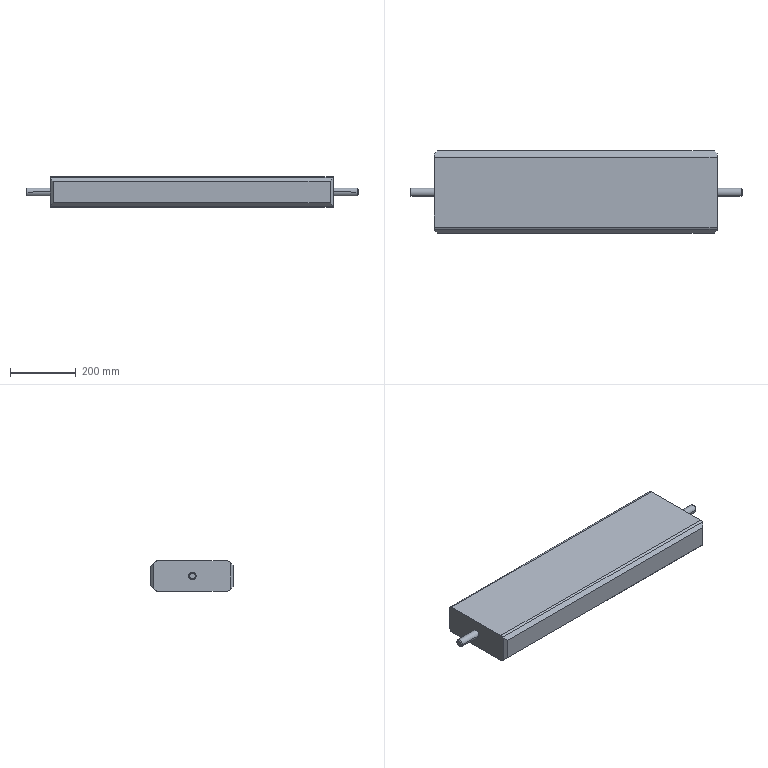Component | SolidWorks | ConnectingBeam-2 | 1 solid | 28 faces | box 1010 x 250 x 92.12 mm | volume 19465625 mm3 | plane 16 | cylinder 8 | cone 4 | commonest cylinder face diameters 24 x4 20 x4
build123d program:
from build123d import *

# Parameters (mm, degrees)
BOSS_EXTRUDE1_DEPTH              = 870
SKETCH2_2_W                      = 12
SKETCH2_2_H                      = 69
SKETCH3_2_W                      = 12
SKETCH3_2_H                      = 71
FILLET1_R                        = 10
CHAMFER1_SIZE2                   = 3
CHAMFER1_SIZE                    = 3
SKETCH2_W                        = 260
SKETCH2_H                        = 120
SKETCH2_R                        = 12
REPAIR_BEAMENDTOWEBLEFT_DEPTH    = 3
SKETCH3_W                        = 260
SKETCH3_H                        = 120
SKETCH3_R                        = 12
REPAIR_BEAMENDTOWEBRIGHT_DEPTH   = 3
REPAIR_BEAMENDCORNERRELIEF_DEPTH = 52.5


with BuildPart() as part:
    # Sketch1 → Boss-Extrude1 (new body)
    with BuildSketch(Plane.XY.offset(454.708)):
        Polygon((127.427, 230.099), (113.427, 216.099), (113.427, 151.98), (127.427, 137.98), (347.427, 137.98), (363.427, 153.98), (363.427, 214.099), (347.427, 230.099), align=None)
    extrude(amount=-BOSS_EXTRUDE1_DEPTH)

    # Sketch2_2 → Revolve1 (revolve)
    with BuildSketch(Plane.XZ.offset(-184.04), mode=Mode.PRIVATE) as revolve1_sk:
        with Locations((243.427, -449.792)):
            Rectangle(SKETCH2_2_W, SKETCH2_2_H)
    revolve(revolve1_sk.sketch.rotate(Axis((237.427, 184.04, -415.292), (0, 0, -1)), 180), axis=Axis((237.427, 184.04, -415.292), (0, 0, -1)))

    # Sketch3_2 → Revolve2 (revolve)
    with BuildSketch(Plane.XZ.offset(-184.04), mode=Mode.PRIVATE) as revolve2_sk:
        with Locations((243.427, 490.208)):
            Rectangle(SKETCH3_2_W, SKETCH3_2_H)
    revolve(revolve2_sk.sketch.rotate(Axis((237.427, 184.04, 525.708), (0, 0, -1)), 180), axis=Axis((237.427, 184.04, 525.708), (0, 0, -1)))

    # Fillet1
    fillet1_edges = [part.edges().sort_by_distance(p)[0] for p in [
        (347.427, 230.099, 19.708),
        (347.427, 137.98, 19.708),
        (127.427, 137.98, 19.708),
        (127.427, 230.099, 19.708),
    ]]
    fillet(fillet1_edges, radius=FILLET1_R)

    # Chamfer1
    chamfer1_edges = [part.edges().sort_by_distance(p)[0] for p in [
        (113.427, 184.04, -415.292),
        (249.427, 184.04, -484.292),
        (363.427, 184.04, -415.292),
        (249.427, 184.04, 525.708),
        (356.891, 220.635, -415.292),
        (237.427, 230.099, 454.708),
        (118.962, 221.635, 454.708),
        (127.742, 229.338, 454.708),
        (347.111, 229.338, 454.708),
        (237.427, 230.099, -415.292),
        (118.962, 221.635, -415.292),
        (127.742, 229.338, -415.292),
        (347.111, 229.338, -415.292),
        (356.891, 220.635, 454.708),
    ]]
    chamfer(chamfer1_edges, length=CHAMFER1_SIZE, length2=CHAMFER1_SIZE2)

    # Sketch2 → Repair_BeamEndToWebLeft (cut, symmetric)
    with BuildSketch(Plane.XY.offset(-413.292)):
        with Locations((237.427, 184.04)):
            Rectangle(SKETCH2_W, SKETCH2_H)
        with Locations(Location((237.427, 184.04, 0), (0, 0, 180))):
            Circle(SKETCH2_R, mode=Mode.SUBTRACT)
    extrude(amount=REPAIR_BEAMENDTOWEBLEFT_DEPTH, both=True, mode=Mode.SUBTRACT)

    # Sketch3 → Repair_BeamEndToWebRight (cut, symmetric)
    with BuildSketch(Plane.XY.offset(452.708)):
        with Locations((237.427, 184.04)):
            Rectangle(SKETCH3_W, SKETCH3_H)
        with Locations(Location((237.427, 184.04, 0), (0, 0, 180))):
            Circle(SKETCH3_R, mode=Mode.SUBTRACT)
    extrude(amount=REPAIR_BEAMENDTOWEBRIGHT_DEPTH, both=True, mode=Mode.SUBTRACT)

    # Sketch4 → Repair_BeamEndCornerRelief (cut, symmetric)
    with BuildSketch(Plane(origin=(0, 184.192, 0), x_dir=(1, 0, 0), z_dir=(0, 1, 0))):
        Polygon((112.427, 411.292), (112.427, 400.292), (123.427, 411.292), align=None)
        Polygon((364.427, 411.292), (364.427, 400.292), (353.427, 411.292), align=None)
        Polygon((112.427, -450.708), (112.427, -439.708), (123.427, -450.708), align=None)
        Polygon((364.427, -450.708), (364.427, -439.708), (353.427, -450.708), align=None)
    extrude(amount=REPAIR_BEAMENDCORNERRELIEF_DEPTH, both=True, mode=Mode.SUBTRACT)


solid = part.part

# Placed as in the assembly
solid = solid.moved(Location((-522.04, 1266.201, -691.692), (90, 90, 0)))
STEP:
#1=COLOUR_RGB('',0.7922,0.8196,0.9333);
#2=FILL_AREA_STYLE_COLOUR('',#1);
#3=FILL_AREA_STYLE('',(#2));
#4=SURFACE_STYLE_FILL_AREA(#3);
#5=SURFACE_SIDE_STYLE('',(#4));
#6=SURFACE_STYLE_USAGE(.BOTH.,#5);
#7=PRESENTATION_STYLE_ASSIGNMENT((#6));
#8=CARTESIAN_POINT('',(0.02629,58.725,-19.986));
#9=VERTEX_POINT('',#8);
#10=CARTESIAN_POINT('',(0.02629,59.67,-19.986));
#11=VERTEX_POINT('',#10);
#12=CARTESIAN_POINT('',(0.02629,59.198,-19.986));
#13=DIRECTION('',(-1.,0.,0.));
#14=DIRECTION('',(0.,1.,0.));
#15=AXIS2_PLACEMENT_3D('',#12,#13,#14);
#16=CIRCLE('',#15,0.4724);
#17=EDGE_CURVE('',#9,#11,#16,.T.);
#18=ORIENTED_EDGE('',*,*,#17,.T.);
#19=CARTESIAN_POINT('',(-2.848,59.67,-19.986));
#20=VERTEX_POINT('',#19);
#21=CARTESIAN_POINT('',(0.1444,59.67,-19.986));
#22=DIRECTION('',(-1.,0.,0.));
#23=VECTOR('',#22,39.37);
#24=LINE('',#21,#23);
#25=EDGE_CURVE('',#11,#20,#24,.T.);
#26=ORIENTED_EDGE('',*,*,#25,.T.);
#27=CARTESIAN_POINT('',(-2.848,58.725,-19.986));
#28=VERTEX_POINT('',#27);
#29=CARTESIAN_POINT('',(-2.848,59.198,-19.986));
#30=DIRECTION('',(1.,0.,0.));
#31=DIRECTION('',(0.,1.,0.));
#32=AXIS2_PLACEMENT_3D('',#29,#30,#31);
#33=CIRCLE('',#32,0.4724);
#34=EDGE_CURVE('',#20,#28,#33,.T.);
#35=ORIENTED_EDGE('',*,*,#34,.T.);
#36=CARTESIAN_POINT('',(0.1444,58.725,-19.986));
#37=DIRECTION('',(-1.,0.,0.));
#38=VECTOR('',#37,39.37);
#39=LINE('',#36,#38);
#40=EDGE_CURVE('',#9,#28,#39,.T.);
#41=ORIENTED_EDGE('',*,*,#40,.F.);
#42=EDGE_LOOP('',(#18,#26,#35,#41));
#43=FACE_OUTER_BOUND('',#42,.T.);
#44=CARTESIAN_POINT('',(0.1444,59.198,-19.986));
#45=DIRECTION('',(-1.,0.,0.));
#46=DIRECTION('',(0.,-1.,0.));
#47=AXIS2_PLACEMENT_3D('',#44,#45,#46);
#48=CYLINDRICAL_SURFACE('',#47,0.4724);
#49=ADVANCED_FACE('',(#43),#48,.T.);
#50=CARTESIAN_POINT('',(0.1444,59.552,-19.986));
#51=VERTEX_POINT('',#50);
#52=CARTESIAN_POINT('',(0.1444,58.844,-19.986));
#53=VERTEX_POINT('',#52);
#54=CARTESIAN_POINT('',(0.1444,59.198,-19.986));
#55=DIRECTION('',(1.,0.,0.));
#56=DIRECTION('',(0.,1.,0.));
#57=AXIS2_PLACEMENT_3D('',#54,#55,#56);
#58=CIRCLE('',#57,0.3543);
#59=EDGE_CURVE('',#51,#53,#58,.T.);
#60=ORIENTED_EDGE('',*,*,#59,.F.);
#61=CARTESIAN_POINT('',(0.02629,59.67,-19.986));
#62=DIRECTION('',(-0.7071,0.7071,0.));
#63=VECTOR('',#62,39.37);
#64=LINE('',#61,#63);
#65=EDGE_CURVE('',#51,#11,#64,.T.);
#66=ORIENTED_EDGE('',*,*,#65,.T.);
#67=ORIENTED_EDGE('',*,*,#17,.F.);
#68=CARTESIAN_POINT('',(0.02629,58.725,-19.986));
#69=DIRECTION('',(-0.7071,-0.7071,0.));
#70=VECTOR('',#69,39.37);
#71=LINE('',#68,#70);
#72=EDGE_CURVE('',#53,#9,#71,.T.);
#73=ORIENTED_EDGE('',*,*,#72,.F.);
#74=EDGE_LOOP('',(#60,#66,#67,#73));
#75=FACE_OUTER_BOUND('',#74,.T.);
#76=CARTESIAN_POINT('',(0.02629,59.198,-19.986));
#77=DIRECTION('',(-1.,0.,0.));
#78=DIRECTION('',(0.,-1.,0.));
#79=AXIS2_PLACEMENT_3D('',#76,#77,#78);
#80=CONICAL_SURFACE('',#79,0.4724,0.7854);
#81=ADVANCED_FACE('',(#75),#80,.T.);
#82=CARTESIAN_POINT('',(-36.706,59.67,-19.986));
#83=VERTEX_POINT('',#82);
#84=CARTESIAN_POINT('',(-36.706,58.725,-19.986));
#85=VERTEX_POINT('',#84);
#86=CARTESIAN_POINT('',(-36.706,59.198,-19.986));
#87=DIRECTION('',(1.,0.,0.));
#88=DIRECTION('',(0.,1.,0.));
#89=AXIS2_PLACEMENT_3D('',#86,#87,#88);
#90=CIRCLE('',#89,0.4724);
#91=EDGE_CURVE('',#83,#85,#90,.T.);
#92=ORIENTED_EDGE('',*,*,#91,.F.);
#93=CARTESIAN_POINT('',(-39.501,59.67,-19.986));
#94=VERTEX_POINT('',#93);
#95=CARTESIAN_POINT('',(-36.903,59.67,-19.986));
#96=DIRECTION('',(-1.,0.,0.));
#97=VECTOR('',#96,39.37);
#98=LINE('',#95,#97);
#99=EDGE_CURVE('',#83,#94,#98,.T.);
#100=ORIENTED_EDGE('',*,*,#99,.T.);
#101=CARTESIAN_POINT('',(-39.501,58.725,-19.986));
#102=VERTEX_POINT('',#101);
#103=CARTESIAN_POINT('',(-39.501,59.198,-19.986));
#104=DIRECTION('',(1.,0.,0.));
#105=DIRECTION('',(0.,-1.,0.));
#106=AXIS2_PLACEMENT_3D('',#103,#104,#105);
#107=CIRCLE('',#106,0.4724);
#108=EDGE_CURVE('',#94,#102,#107,.T.);
#109=ORIENTED_EDGE('',*,*,#108,.T.);
#110=CARTESIAN_POINT('',(-36.903,58.725,-19.986));
#111=DIRECTION('',(-1.,0.,0.));
#112=VECTOR('',#111,39.37);
#113=LINE('',#110,#112);
#114=EDGE_CURVE('',#85,#102,#113,.T.);
#115=ORIENTED_EDGE('',*,*,#114,.F.);
#116=EDGE_LOOP('',(#92,#100,#109,#115));
#117=FACE_OUTER_BOUND('',#116,.T.);
#118=CARTESIAN_POINT('',(-36.903,59.198,-19.986));
#119=DIRECTION('',(-1.,0.,0.));
#120=DIRECTION('',(0.,-1.,0.));
#121=AXIS2_PLACEMENT_3D('',#118,#119,#120);
#122=CYLINDRICAL_SURFACE('',#121,0.4724);
#123=ADVANCED_FACE('',(#117),#122,.T.);
#124=CARTESIAN_POINT('',(-39.619,58.844,-19.986));
#125=VERTEX_POINT('',#124);
#126=CARTESIAN_POINT('',(-39.619,59.552,-19.986));
#127=VERTEX_POINT('',#126);
#128=CARTESIAN_POINT('',(-39.619,59.198,-19.986));
#129=DIRECTION('',(-1.,0.,0.));
#130=DIRECTION('',(0.,-1.,0.));
#131=AXIS2_PLACEMENT_3D('',#128,#129,#130);
#132=CIRCLE('',#131,0.3543);
#133=EDGE_CURVE('',#125,#127,#132,.T.);
#134=ORIENTED_EDGE('',*,*,#133,.F.);
#135=CARTESIAN_POINT('',(-39.619,58.844,-19.986));
#136=DIRECTION('',(0.7071,-0.7071,0.));
#137=VECTOR('',#136,39.37);
#138=LINE('',#135,#137);
#139=EDGE_CURVE('',#125,#102,#138,.T.);
#140=ORIENTED_EDGE('',*,*,#139,.T.);
#141=ORIENTED_EDGE('',*,*,#108,.F.);
#142=CARTESIAN_POINT('',(-39.619,59.552,-19.986));
#143=DIRECTION('',(0.7071,0.7071,0.));
#144=VECTOR('',#143,39.37);
#145=LINE('',#142,#144);
#146=EDGE_CURVE('',#127,#94,#145,.T.);
#147=ORIENTED_EDGE('',*,*,#146,.F.);
#148=EDGE_LOOP('',(#134,#140,#141,#147));
#149=FACE_OUTER_BOUND('',#148,.T.);
#150=CARTESIAN_POINT('',(-39.619,59.198,-19.986));
#151=DIRECTION('',(1.,0.,0.));
#152=DIRECTION('',(0.,1.,0.));
#153=AXIS2_PLACEMENT_3D('',#150,#151,#152);
#154=CONICAL_SURFACE('',#153,0.3543,0.7854);
#155=ADVANCED_FACE('',(#149),#154,.T.);
#156=CARTESIAN_POINT('',(-36.706,55.03,-18.173));
#157=VERTEX_POINT('',#156);
#158=CARTESIAN_POINT('',(-2.848,55.03,-18.173));
#159=VERTEX_POINT('',#158);
#160=CARTESIAN_POINT('',(-36.903,55.03,-18.173));
#161=DIRECTION('',(1.,0.,0.));
#162=VECTOR('',#161,39.37);
#163=LINE('',#160,#162);
#164=EDGE_CURVE('',#157,#159,#163,.T.);
#165=ORIENTED_EDGE('',*,*,#164,.T.);
#166=CARTESIAN_POINT('',(-2.848,63.366,-18.173));
#167=VERTEX_POINT('',#166);
#168=CARTESIAN_POINT('',(-2.848,63.529,-18.173));
#169=DIRECTION('',(0.,1.,0.));
#170=VECTOR('',#169,39.37);
#171=LINE('',#168,#170);
#172=EDGE_CURVE('',#159,#167,#171,.T.);
#173=ORIENTED_EDGE('',*,*,#172,.T.);
#174=CARTESIAN_POINT('',(-36.706,63.366,-18.173));
#175=VERTEX_POINT('',#174);
#176=CARTESIAN_POINT('',(-36.903,63.366,-18.173));
#177=DIRECTION('',(-1.,0.,0.));
#178=VECTOR('',#177,39.37);
#179=LINE('',#176,#178);
#180=EDGE_CURVE('',#167,#175,#179,.T.);
#181=ORIENTED_EDGE('',*,*,#180,.T.);
#182=CARTESIAN_POINT('',(-36.706,63.529,-18.173));
#183=DIRECTION('',(0.,1.,0.));
#184=VECTOR('',#183,39.37);
#185=LINE('',#182,#184);
#186=EDGE_CURVE('',#157,#175,#185,.T.);
#187=ORIENTED_EDGE('',*,*,#186,.F.);
#188=EDGE_LOOP('',(#165,#173,#181,#187));
#189=FACE_OUTER_BOUND('',#188,.T.);
#190=CARTESIAN_POINT('',(-36.903,63.529,-18.173));
#191=DIRECTION('',(0.,0.,1.));
#192=DIRECTION('',(1.,0.,0.));
#193=AXIS2_PLACEMENT_3D('',#190,#191,#192);
#194=PLANE('',#193);
#195=ADVANCED_FACE('',(#189),#194,.T.);
#196=CARTESIAN_POINT('',(-36.706,63.804,-18.449));
#197=VERTEX_POINT('',#196);
#198=CARTESIAN_POINT('',(-36.352,64.159,-18.803));
#199=VERTEX_POINT('',#198);
#200=CARTESIAN_POINT('',(-36.535,63.975,-18.619));
#201=DIRECTION('',(0.5774,0.5774,-0.5774));
#202=VECTOR('',#201,39.37);
#203=LINE('',#200,#202);
#204=EDGE_CURVE('',#197,#199,#203,.T.);
#205=ORIENTED_EDGE('',*,*,#204,.F.);
#206=CARTESIAN_POINT('',(-36.706,63.644,-18.288));
#207=VERTEX_POINT('',#206);
#208=CARTESIAN_POINT('',(-36.706,64.159,-18.803));
#209=DIRECTION('',(0.,0.7071,-0.7071));
#210=VECTOR('',#209,39.37);
#211=LINE('',#208,#210);
#212=EDGE_CURVE('',#207,#197,#211,.T.);
#213=ORIENTED_EDGE('',*,*,#212,.F.);
#214=CARTESIAN_POINT('',(-2.848,63.644,-18.288));
#215=VERTEX_POINT('',#214);
#216=CARTESIAN_POINT('',(-36.903,63.644,-18.288));
#217=DIRECTION('',(1.,0.,0.));
#218=VECTOR('',#217,39.37);
#219=LINE('',#216,#218);
#220=EDGE_CURVE('',#207,#215,#219,.T.);
#221=ORIENTED_EDGE('',*,*,#220,.T.);
#222=CARTESIAN_POINT('',(-2.848,63.804,-18.449));
#223=VERTEX_POINT('',#222);
#224=CARTESIAN_POINT('',(-2.848,64.159,-18.803));
#225=DIRECTION('',(0.,0.7071,-0.7071));
#226=VECTOR('',#225,39.37);
#227=LINE('',#224,#226);
#228=EDGE_CURVE('',#215,#223,#227,.T.);
#229=ORIENTED_EDGE('',*,*,#228,.T.);
#230=CARTESIAN_POINT('',(-3.202,64.159,-18.803));
#231=VERTEX_POINT('',#230);
#232=CARTESIAN_POINT('',(-14.436,75.392,-30.036));
#233=DIRECTION('',(0.5774,-0.5774,0.5774));
#234=VECTOR('',#233,39.37);
#235=LINE('',#232,#234);
#236=EDGE_CURVE('',#231,#223,#235,.T.);
#237=ORIENTED_EDGE('',*,*,#236,.F.);
#238=CARTESIAN_POINT('',(-36.903,64.159,-18.803));
#239=DIRECTION('',(1.,0.,0.));
#240=VECTOR('',#239,39.37);
#241=LINE('',#238,#240);
#242=EDGE_CURVE('',#199,#231,#241,.T.);
#243=ORIENTED_EDGE('',*,*,#242,.F.);
#244=EDGE_LOOP('',(#205,#213,#221,#229,#237,#243));
#245=FACE_OUTER_BOUND('',#244,.T.);
#246=CARTESIAN_POINT('',(-36.903,64.159,-18.803));
#247=DIRECTION('',(0.,0.7071,0.7071));
#248=DIRECTION('',(0.,-0.7071,0.7071));
#249=AXIS2_PLACEMENT_3D('',#246,#247,#248);
#250=PLANE('',#249);
#251=ADVANCED_FACE('',(#245),#250,.T.);
#252=CARTESIAN_POINT('',(-36.352,64.159,-21.17));
#253=VERTEX_POINT('',#252);
#254=CARTESIAN_POINT('',(-36.352,64.159,-21.17));
#255=DIRECTION('',(0.,0.,-1.));
#256=VECTOR('',#255,39.37);
#257=LINE('',#254,#256);
#258=EDGE_CURVE('',#199,#253,#257,.T.);
#259=ORIENTED_EDGE('',*,*,#258,.F.);
#260=ORIENTED_EDGE('',*,*,#242,.T.);
#261=CARTESIAN_POINT('',(-3.202,64.159,-21.17));
#262=VERTEX_POINT('',#261);
#263=CARTESIAN_POINT('',(-3.202,64.159,-21.17));
#264=DIRECTION('',(0.,0.,1.));
#265=VECTOR('',#264,39.37);
#266=LINE('',#263,#265);
#267=EDGE_CURVE('',#262,#231,#266,.T.);
#268=ORIENTED_EDGE('',*,*,#267,.F.);
#269=CARTESIAN_POINT('',(-36.903,64.159,-21.17));
#270=DIRECTION('',(1.,0.,0.));
#271=VECTOR('',#270,39.37);
#272=LINE('',#269,#271);
#273=EDGE_CURVE('',#253,#262,#272,.T.);
#274=ORIENTED_EDGE('',*,*,#273,.F.);
#275=EDGE_LOOP('',(#259,#260,#268,#274));
#276=FACE_OUTER_BOUND('',#275,.T.);
#277=CARTESIAN_POINT('',(-36.903,64.159,-21.17));
#278=DIRECTION('',(0.,1.,0.));
#279=DIRECTION('',(-1.,0.,0.));
#280=AXIS2_PLACEMENT_3D('',#277,#278,#279);
#281=PLANE('',#280);
#282=ADVANCED_FACE('',(#276),#281,.T.);
#283=CARTESIAN_POINT('',(-36.706,63.804,-21.524));
#284=VERTEX_POINT('',#283);
#285=CARTESIAN_POINT('',(-36.955,63.555,-21.773));
#286=DIRECTION('',(-0.5774,-0.5774,-0.5774));
#287=VECTOR('',#286,39.37);
#288=LINE('',#285,#287);
#289=EDGE_CURVE('',#253,#284,#288,.T.);
#290=ORIENTED_EDGE('',*,*,#289,.F.);
#291=ORIENTED_EDGE('',*,*,#273,.T.);
#292=CARTESIAN_POINT('',(-2.848,63.804,-21.524));
#293=VERTEX_POINT('',#292);
#294=CARTESIAN_POINT('',(-14.016,74.972,-10.356));
#295=DIRECTION('',(-0.5774,0.5774,0.5774));
#296=VECTOR('',#295,39.37);
#297=LINE('',#294,#296);
#298=EDGE_CURVE('',#293,#262,#297,.T.);
#299=ORIENTED_EDGE('',*,*,#298,.F.);
#300=CARTESIAN_POINT('',(-2.848,63.644,-21.684));
#301=VERTEX_POINT('',#300);
#302=CARTESIAN_POINT('',(-2.848,63.529,-21.8));
#303=DIRECTION('',(0.,-0.7071,-0.7071));
#304=VECTOR('',#303,39.37);
#305=LINE('',#302,#304);
#306=EDGE_CURVE('',#293,#301,#305,.T.);
#307=ORIENTED_EDGE('',*,*,#306,.T.);
#308=CARTESIAN_POINT('',(-36.706,63.644,-21.684));
#309=VERTEX_POINT('',#308);
#310=CARTESIAN_POINT('',(-36.903,63.644,-21.684));
#311=DIRECTION('',(-1.,0.,0.));
#312=VECTOR('',#311,39.37);
#313=LINE('',#310,#312);
#314=EDGE_CURVE('',#301,#309,#313,.T.);
#315=ORIENTED_EDGE('',*,*,#314,.T.);
#316=CARTESIAN_POINT('',(-36.706,63.529,-21.8));
#317=DIRECTION('',(0.,-0.7071,-0.7071));
#318=VECTOR('',#317,39.37);
#319=LINE('',#316,#318);
#320=EDGE_CURVE('',#284,#309,#319,.T.);
#321=ORIENTED_EDGE('',*,*,#320,.F.);
#322=EDGE_LOOP('',(#290,#291,#299,#307,#315,#321));
#323=FACE_OUTER_BOUND('',#322,.T.);
#324=CARTESIAN_POINT('',(-36.903,63.529,-21.8));
#325=DIRECTION('',(0.,0.7071,-0.7071));
#326=DIRECTION('',(0.,0.7071,0.7071));
#327=AXIS2_PLACEMENT_3D('',#324,#325,#326);
#328=PLANE('',#327);
#329=ADVANCED_FACE('',(#323),#328,.T.);
#330=CARTESIAN_POINT('',(-36.706,63.366,-21.8));
#331=VERTEX_POINT('',#330);
#332=CARTESIAN_POINT('',(-2.848,63.366,-21.8));
#333=VERTEX_POINT('',#332);
#334=CARTESIAN_POINT('',(-36.903,63.366,-21.8));
#335=DIRECTION('',(1.,0.,0.));
#336=VECTOR('',#335,39.37);
#337=LINE('',#334,#336);
#338=EDGE_CURVE('',#331,#333,#337,.T.);
#339=ORIENTED_EDGE('',*,*,#338,.T.);
#340=CARTESIAN_POINT('',(-2.848,55.03,-21.8));
#341=VERTEX_POINT('',#340);
#342=CARTESIAN_POINT('',(-2.848,54.867,-21.8));
#343=DIRECTION('',(0.,-1.,-0.));
#344=VECTOR('',#343,39.37);
#345=LINE('',#342,#344);
#346=EDGE_CURVE('',#333,#341,#345,.T.);
#347=ORIENTED_EDGE('',*,*,#346,.T.);
#348=CARTESIAN_POINT('',(-36.706,55.03,-21.8));
#349=VERTEX_POINT('',#348);
#350=CARTESIAN_POINT('',(-36.903,55.03,-21.8));
#351=DIRECTION('',(-1.,0.,0.));
#352=VECTOR('',#351,39.37);
#353=LINE('',#350,#352);
#354=EDGE_CURVE('',#341,#349,#353,.T.);
#355=ORIENTED_EDGE('',*,*,#354,.T.);
#356=CARTESIAN_POINT('',(-36.706,54.867,-21.8));
#357=DIRECTION('',(0.,-1.,-0.));
#358=VECTOR('',#357,39.37);
#359=LINE('',#356,#358);
#360=EDGE_CURVE('',#331,#349,#359,.T.);
#361=ORIENTED_EDGE('',*,*,#360,.F.);
#362=EDGE_LOOP('',(#339,#347,#355,#361));
#363=FACE_OUTER_BOUND('',#362,.T.);
#364=CARTESIAN_POINT('',(-36.903,54.867,-21.8));
#365=DIRECTION('',(0.,0.,-1.));
#366=DIRECTION('',(0.,1.,0.));
#367=AXIS2_PLACEMENT_3D('',#364,#365,#366);
#368=PLANE('',#367);
#369=ADVANCED_FACE('',(#363),#368,.T.);
#370=CARTESIAN_POINT('',(-3.202,54.316,-21.248));
#371=VERTEX_POINT('',#370);
#372=CARTESIAN_POINT('',(-2.848,54.67,-21.603));
#373=VERTEX_POINT('',#372);
#374=CARTESIAN_POINT('',(-14.436,43.082,-10.015));
#375=DIRECTION('',(0.5774,0.5774,-0.5774));
#376=VECTOR('',#375,39.37);
#377=LINE('',#374,#376);
#378=EDGE_CURVE('',#371,#373,#377,.T.);
#379=ORIENTED_EDGE('',*,*,#378,.F.);
#380=CARTESIAN_POINT('',(-36.352,54.316,-21.248));
#381=VERTEX_POINT('',#380);
#382=CARTESIAN_POINT('',(-36.903,54.316,-21.248));
#383=DIRECTION('',(1.,0.,0.));
#384=VECTOR('',#383,39.37);
#385=LINE('',#382,#384);
#386=EDGE_CURVE('',#381,#371,#385,.T.);
#387=ORIENTED_EDGE('',*,*,#386,.F.);
#388=CARTESIAN_POINT('',(-36.706,54.67,-21.603));
#389=VERTEX_POINT('',#388);
#390=CARTESIAN_POINT('',(-36.535,54.5,-21.432));
#391=DIRECTION('',(0.5774,-0.5774,0.5774));
#392=VECTOR('',#391,39.37);
#393=LINE('',#390,#392);
#394=EDGE_CURVE('',#389,#381,#393,.T.);
#395=ORIENTED_EDGE('',*,*,#394,.F.);
#396=CARTESIAN_POINT('',(-36.706,54.752,-21.684));
#397=VERTEX_POINT('',#396);
#398=CARTESIAN_POINT('',(-36.706,54.316,-21.248));
#399=DIRECTION('',(0.,-0.7071,0.7071));
#400=VECTOR('',#399,39.37);
#401=LINE('',#398,#400);
#402=EDGE_CURVE('',#397,#389,#401,.T.);
#403=ORIENTED_EDGE('',*,*,#402,.F.);
#404=CARTESIAN_POINT('',(-2.848,54.752,-21.684));
#405=VERTEX_POINT('',#404);
#406=CARTESIAN_POINT('',(-36.903,54.752,-21.684));
#407=DIRECTION('',(1.,0.,0.));
#408=VECTOR('',#407,39.37);
#409=LINE('',#406,#408);
#410=EDGE_CURVE('',#397,#405,#409,.T.);
#411=ORIENTED_EDGE('',*,*,#410,.T.);
#412=CARTESIAN_POINT('',(-2.848,54.316,-21.248));
#413=DIRECTION('',(0.,-0.7071,0.7071));
#414=VECTOR('',#413,39.37);
#415=LINE('',#412,#414);
#416=EDGE_CURVE('',#405,#373,#415,.T.);
#417=ORIENTED_EDGE('',*,*,#416,.T.);
#418=EDGE_LOOP('',(#379,#387,#395,#403,#411,#417));
#419=FACE_OUTER_BOUND('',#418,.T.);
#420=CARTESIAN_POINT('',(-36.903,54.316,-21.248));
#421=DIRECTION('',(0.,-0.7071,-0.7071));
#422=DIRECTION('',(0.,0.7071,-0.7071));
#423=AXIS2_PLACEMENT_3D('',#420,#421,#422);
#424=PLANE('',#423);
#425=ADVANCED_FACE('',(#419),#424,.T.);
#426=CARTESIAN_POINT('',(-3.202,54.316,-18.724));
#427=VERTEX_POINT('',#426);
#428=CARTESIAN_POINT('',(-3.202,54.316,-18.724));
#429=DIRECTION('',(0.,0.,-1.));
#430=VECTOR('',#429,39.37);
#431=LINE('',#428,#430);
#432=EDGE_CURVE('',#427,#371,#431,.T.);
#433=ORIENTED_EDGE('',*,*,#432,.F.);
#434=CARTESIAN_POINT('',(-36.352,54.316,-18.724));
#435=VERTEX_POINT('',#434);
#436=CARTESIAN_POINT('',(-36.903,54.316,-18.724));
#437=DIRECTION('',(1.,0.,0.));
#438=VECTOR('',#437,39.37);
#439=LINE('',#436,#438);
#440=EDGE_CURVE('',#435,#427,#439,.T.);
#441=ORIENTED_EDGE('',*,*,#440,.F.);
#442=CARTESIAN_POINT('',(-36.352,54.316,-18.724));
#443=DIRECTION('',(0.,0.,1.));
#444=VECTOR('',#443,39.37);
#445=LINE('',#442,#444);
#446=EDGE_CURVE('',#381,#435,#445,.T.);
#447=ORIENTED_EDGE('',*,*,#446,.F.);
#448=ORIENTED_EDGE('',*,*,#386,.T.);
#449=EDGE_LOOP('',(#433,#441,#447,#448));
#450=FACE_OUTER_BOUND('',#449,.T.);
#451=CARTESIAN_POINT('',(-36.903,54.316,-18.724));
#452=DIRECTION('',(0.,-1.,0.));
#453=DIRECTION('',(1.,0.,0.));
#454=AXIS2_PLACEMENT_3D('',#451,#452,#453);
#455=PLANE('',#454);
#456=ADVANCED_FACE('',(#450),#455,.T.);
#457=CARTESIAN_POINT('',(-2.848,54.67,-18.37));
#458=VERTEX_POINT('',#457);
#459=CARTESIAN_POINT('',(-14.068,43.45,-29.59));
#460=DIRECTION('',(-0.5774,-0.5774,-0.5774));
#461=VECTOR('',#460,39.37);
#462=LINE('',#459,#461);
#463=EDGE_CURVE('',#458,#427,#462,.T.);
#464=ORIENTED_EDGE('',*,*,#463,.F.);
#465=CARTESIAN_POINT('',(-2.848,54.752,-18.288));
#466=VERTEX_POINT('',#465);
#467=CARTESIAN_POINT('',(-2.848,54.867,-18.173));
#468=DIRECTION('',(0.,0.7071,0.7071));
#469=VECTOR('',#468,39.37);
#470=LINE('',#467,#469);
#471=EDGE_CURVE('',#458,#466,#470,.T.);
#472=ORIENTED_EDGE('',*,*,#471,.T.);
#473=CARTESIAN_POINT('',(-36.706,54.752,-18.288));
#474=VERTEX_POINT('',#473);
#475=CARTESIAN_POINT('',(-36.903,54.752,-18.288));
#476=DIRECTION('',(-1.,0.,0.));
#477=VECTOR('',#476,39.37);
#478=LINE('',#475,#477);
#479=EDGE_CURVE('',#466,#474,#478,.T.);
#480=ORIENTED_EDGE('',*,*,#479,.T.);
#481=CARTESIAN_POINT('',(-36.706,54.67,-18.37));
#482=VERTEX_POINT('',#481);
#483=CARTESIAN_POINT('',(-36.706,54.867,-18.173));
#484=DIRECTION('',(0.,0.7071,0.7071));
#485=VECTOR('',#484,39.37);
#486=LINE('',#483,#485);
#487=EDGE_CURVE('',#482,#474,#486,.T.);
#488=ORIENTED_EDGE('',*,*,#487,.F.);
#489=CARTESIAN_POINT('',(-36.903,54.867,-18.173));
#490=DIRECTION('',(-0.5774,0.5774,0.5774));
#491=VECTOR('',#490,39.37);
#492=LINE('',#489,#491);
#493=EDGE_CURVE('',#435,#482,#492,.T.);
#494=ORIENTED_EDGE('',*,*,#493,.F.);
#495=ORIENTED_EDGE('',*,*,#440,.T.);
#496=EDGE_LOOP('',(#464,#472,#480,#488,#494,#495));
#497=FACE_OUTER_BOUND('',#496,.T.);
#498=CARTESIAN_POINT('',(-36.903,54.867,-18.173));
#499=DIRECTION('',(0.,-0.7071,0.7071));
#500=DIRECTION('',(0.,-0.7071,-0.7071));
#501=AXIS2_PLACEMENT_3D('',#498,#499,#500);
#502=PLANE('',#501);
#503=ADVANCED_FACE('',(#497),#502,.T.);
#504=ORIENTED_EDGE('',*,*,#314,.F.);
#505=CARTESIAN_POINT('',(-2.848,63.366,-21.406));
#506=DIRECTION('',(-1.,0.,0.));
#507=DIRECTION('',(0.,1.,0.));
#508=AXIS2_PLACEMENT_3D('',#505,#506,#507);
#509=CIRCLE('',#508,0.3937);
#510=EDGE_CURVE('',#301,#333,#509,.T.);
#511=ORIENTED_EDGE('',*,*,#510,.T.);
#512=ORIENTED_EDGE('',*,*,#338,.F.);
#513=CARTESIAN_POINT('',(-36.706,63.366,-21.406));
#514=DIRECTION('',(-1.,0.,0.));
#515=DIRECTION('',(0.,1.,0.));
#516=AXIS2_PLACEMENT_3D('',#513,#514,#515);
#517=CIRCLE('',#516,0.3937);
#518=EDGE_CURVE('',#309,#331,#517,.T.);
#519=ORIENTED_EDGE('',*,*,#518,.F.);
#520=EDGE_LOOP('',(#504,#511,#512,#519));
#521=FACE_OUTER_BOUND('',#520,.T.);
#522=CARTESIAN_POINT('',(-36.903,63.366,-21.406));
#523=DIRECTION('',(1.,0.,0.));
#524=DIRECTION('',(0.,1.,0.));
#525=AXIS2_PLACEMENT_3D('',#522,#523,#524);
#526=CYLINDRICAL_SURFACE('',#525,0.3937);
#527=ADVANCED_FACE('',(#521),#526,.T.);
#528=ORIENTED_EDGE('',*,*,#354,.F.);
#529=CARTESIAN_POINT('',(-2.848,55.03,-21.406));
#530=DIRECTION('',(-1.,0.,0.));
#531=DIRECTION('',(0.,1.,0.));
#532=AXIS2_PLACEMENT_3D('',#529,#530,#531);
#533=CIRCLE('',#532,0.3937);
#534=EDGE_CURVE('',#341,#405,#533,.T.);
#535=ORIENTED_EDGE('',*,*,#534,.T.);
#536=ORIENTED_EDGE('',*,*,#410,.F.);
#537=CARTESIAN_POINT('',(-36.706,55.03,-21.406));
#538=DIRECTION('',(-1.,0.,0.));
#539=DIRECTION('',(0.,1.,0.));
#540=AXIS2_PLACEMENT_3D('',#537,#538,#539);
#541=CIRCLE('',#540,0.3937);
#542=EDGE_CURVE('',#349,#397,#541,.T.);
#543=ORIENTED_EDGE('',*,*,#542,.F.);
#544=EDGE_LOOP('',(#528,#535,#536,#543));
#545=FACE_OUTER_BOUND('',#544,.T.);
#546=CARTESIAN_POINT('',(-36.903,55.03,-21.406));
#547=DIRECTION('',(1.,0.,0.));
#548=DIRECTION('',(0.,1.,0.));
#549=AXIS2_PLACEMENT_3D('',#546,#547,#548);
#550=CYLINDRICAL_SURFACE('',#549,0.3937);
#551=ADVANCED_FACE('',(#545),#550,.T.);
#552=ORIENTED_EDGE('',*,*,#180,.F.);
#553=CARTESIAN_POINT('',(-2.848,63.366,-18.567));
#554=DIRECTION('',(-1.,0.,0.));
#555=DIRECTION('',(0.,1.,-0.));
#556=AXIS2_PLACEMENT_3D('',#553,#554,#555);
#557=CIRCLE('',#556,0.3937);
#558=EDGE_CURVE('',#167,#215,#557,.T.);
#559=ORIENTED_EDGE('',*,*,#558,.T.);
#560=ORIENTED_EDGE('',*,*,#220,.F.);
#561=CARTESIAN_POINT('',(-36.706,63.366,-18.567));
#562=DIRECTION('',(-1.,0.,0.));
#563=DIRECTION('',(0.,1.,-0.));
#564=AXIS2_PLACEMENT_3D('',#561,#562,#563);
#565=CIRCLE('',#564,0.3937);
#566=EDGE_CURVE('',#175,#207,#565,.T.);
#567=ORIENTED_EDGE('',*,*,#566,.F.);
#568=EDGE_LOOP('',(#552,#559,#560,#567));
#569=FACE_OUTER_BOUND('',#568,.T.);
#570=CARTESIAN_POINT('',(-36.903,63.366,-18.567));
#571=DIRECTION('',(1.,0.,0.));
#572=DIRECTION('',(0.,1.,0.));
#573=AXIS2_PLACEMENT_3D('',#570,#571,#572);
#574=CYLINDRICAL_SURFACE('',#573,0.3937);
#575=ADVANCED_FACE('',(#569),#574,.T.);
#576=ORIENTED_EDGE('',*,*,#479,.F.);
#577=CARTESIAN_POINT('',(-2.848,55.03,-18.567));
#578=DIRECTION('',(-1.,0.,0.));
#579=DIRECTION('',(0.,1.,-0.));
#580=AXIS2_PLACEMENT_3D('',#577,#578,#579);
#581=CIRCLE('',#580,0.3937);
#582=EDGE_CURVE('',#466,#159,#581,.T.);
#583=ORIENTED_EDGE('',*,*,#582,.T.);
#584=ORIENTED_EDGE('',*,*,#164,.F.);
#585=CARTESIAN_POINT('',(-36.706,55.03,-18.567));
#586=DIRECTION('',(-1.,0.,0.));
#587=DIRECTION('',(0.,1.,-0.));
#588=AXIS2_PLACEMENT_3D('',#585,#586,#587);
#589=CIRCLE('',#588,0.3937);
#590=EDGE_CURVE('',#474,#157,#589,.T.);
#591=ORIENTED_EDGE('',*,*,#590,.F.);
#592=EDGE_LOOP('',(#576,#583,#584,#591));
#593=FACE_OUTER_BOUND('',#592,.T.);
#594=CARTESIAN_POINT('',(-36.903,55.03,-18.567));
#595=DIRECTION('',(1.,0.,0.));
#596=DIRECTION('',(0.,1.,0.));
#597=AXIS2_PLACEMENT_3D('',#594,#595,#596);
#598=CYLINDRICAL_SURFACE('',#597,0.3937);
#599=ADVANCED_FACE('',(#593),#598,.T.);
#600=ORIENTED_EDGE('',*,*,#212,.T.);
#601=CARTESIAN_POINT('',(-36.706,63.804,-27.232));
#602=DIRECTION('',(0.,0.,-1.));
#603=VECTOR('',#602,39.37);
#604=LINE('',#601,#603);
#605=EDGE_CURVE('',#197,#284,#604,.T.);
#606=ORIENTED_EDGE('',*,*,#605,.T.);
#607=ORIENTED_EDGE('',*,*,#320,.T.);
#608=ORIENTED_EDGE('',*,*,#518,.T.);
#609=ORIENTED_EDGE('',*,*,#360,.T.);
#610=ORIENTED_EDGE('',*,*,#542,.T.);
#611=ORIENTED_EDGE('',*,*,#402,.T.);
#612=CARTESIAN_POINT('',(-36.706,54.67,-27.232));
#613=DIRECTION('',(0.,0.,1.));
#614=VECTOR('',#613,39.37);
#615=LINE('',#612,#614);
#616=EDGE_CURVE('',#389,#482,#615,.T.);
#617=ORIENTED_EDGE('',*,*,#616,.T.);
#618=ORIENTED_EDGE('',*,*,#487,.T.);
#619=ORIENTED_EDGE('',*,*,#590,.T.);
#620=ORIENTED_EDGE('',*,*,#186,.T.);
#621=ORIENTED_EDGE('',*,*,#566,.T.);
#622=EDGE_LOOP('',(#600,#606,#607,#608,#609,#610,#611,#617,#618,#619,#620,#621));
#623=FACE_OUTER_BOUND('',#622,.T.);
#624=CARTESIAN_POINT('',(-36.706,59.198,-19.986));
#625=DIRECTION('',(1.,0.,0.));
#626=DIRECTION('',(0.,1.,0.));
#627=AXIS2_PLACEMENT_3D('',#624,#625,#626);
#628=CIRCLE('',#627,0.4724);
#629=EDGE_CURVE('',#85,#83,#628,.T.);
#630=ORIENTED_EDGE('',*,*,#629,.T.);
#631=ORIENTED_EDGE('',*,*,#91,.T.);
#632=EDGE_LOOP('',(#630,#631));
#633=FACE_BOUND('',#632,.T.);
#634=CARTESIAN_POINT('',(-36.706,49.85,-27.232));
#635=DIRECTION('',(1.,0.,0.));
#636=DIRECTION('',(0.,1.,0.));
#637=AXIS2_PLACEMENT_3D('',#634,#635,#636);
#638=PLANE('',#637);
#639=ADVANCED_FACE('',(#623,#633),#638,.F.);
#640=CARTESIAN_POINT('',(-39.619,59.198,-19.986));
#641=DIRECTION('',(-1.,0.,0.));
#642=DIRECTION('',(0.,-1.,0.));
#643=AXIS2_PLACEMENT_3D('',#640,#641,#642);
#644=CIRCLE('',#643,0.3543);
#645=EDGE_CURVE('',#127,#125,#644,.T.);
#646=ORIENTED_EDGE('',*,*,#645,.T.);
#647=ORIENTED_EDGE('',*,*,#133,.T.);
#648=EDGE_LOOP('',(#646,#647));
#649=FACE_OUTER_BOUND('',#648,.T.);
#650=CARTESIAN_POINT('',(-39.619,59.198,-19.986));
#651=DIRECTION('',(-1.,0.,0.));
#652=DIRECTION('',(0.,-1.,0.));
#653=AXIS2_PLACEMENT_3D('',#650,#651,#652);
#654=PLANE('',#653);
#655=ADVANCED_FACE('',(#649),#654,.T.);
#656=ORIENTED_EDGE('',*,*,#139,.F.);
#657=ORIENTED_EDGE('',*,*,#645,.F.);
#658=ORIENTED_EDGE('',*,*,#146,.T.);
#659=CARTESIAN_POINT('',(-39.501,59.198,-19.986));
#660=DIRECTION('',(1.,0.,0.));
#661=DIRECTION('',(0.,-1.,0.));
#662=AXIS2_PLACEMENT_3D('',#659,#660,#661);
#663=CIRCLE('',#662,0.4724);
#664=EDGE_CURVE('',#102,#94,#663,.T.);
#665=ORIENTED_EDGE('',*,*,#664,.F.);
#666=EDGE_LOOP('',(#656,#657,#658,#665));
#667=FACE_OUTER_BOUND('',#666,.T.);
#668=CARTESIAN_POINT('',(-39.619,59.198,-19.986));
#669=DIRECTION('',(1.,0.,0.));
#670=DIRECTION('',(0.,1.,0.));
#671=AXIS2_PLACEMENT_3D('',#668,#669,#670);
#672=CONICAL_SURFACE('',#671,0.3543,0.7854);
#673=ADVANCED_FACE('',(#667),#672,.T.);
#674=ORIENTED_EDGE('',*,*,#99,.F.);
#675=ORIENTED_EDGE('',*,*,#629,.F.);
#676=ORIENTED_EDGE('',*,*,#114,.T.);
#677=ORIENTED_EDGE('',*,*,#664,.T.);
#678=EDGE_LOOP('',(#674,#675,#676,#677));
#679=FACE_OUTER_BOUND('',#678,.T.);
#680=CARTESIAN_POINT('',(-36.903,59.198,-19.986));
#681=DIRECTION('',(-1.,0.,0.));
#682=DIRECTION('',(0.,-1.,0.));
#683=AXIS2_PLACEMENT_3D('',#680,#681,#682);
#684=CYLINDRICAL_SURFACE('',#683,0.4724);
#685=ADVANCED_FACE('',(#679),#684,.T.);
#686=CARTESIAN_POINT('',(-2.848,54.67,-27.232));
#687=DIRECTION('',(0.,0.,1.));
#688=VECTOR('',#687,39.37);
#689=LINE('',#686,#688);
#690=EDGE_CURVE('',#373,#458,#689,.T.);
#691=ORIENTED_EDGE('',*,*,#690,.F.);
#692=ORIENTED_EDGE('',*,*,#416,.F.);
#693=ORIENTED_EDGE('',*,*,#534,.F.);
#694=ORIENTED_EDGE('',*,*,#346,.F.);
#695=ORIENTED_EDGE('',*,*,#510,.F.);
#696=ORIENTED_EDGE('',*,*,#306,.F.);
#697=CARTESIAN_POINT('',(-2.848,63.804,-27.232));
#698=DIRECTION('',(0.,0.,-1.));
#699=VECTOR('',#698,39.37);
#700=LINE('',#697,#699);
#701=EDGE_CURVE('',#223,#293,#700,.T.);
#702=ORIENTED_EDGE('',*,*,#701,.F.);
#703=ORIENTED_EDGE('',*,*,#228,.F.);
#704=ORIENTED_EDGE('',*,*,#558,.F.);
#705=ORIENTED_EDGE('',*,*,#172,.F.);
#706=ORIENTED_EDGE('',*,*,#582,.F.);
#707=ORIENTED_EDGE('',*,*,#471,.F.);
#708=EDGE_LOOP('',(#691,#692,#693,#694,#695,#696,#702,#703,#704,#705,#706,#707));
#709=FACE_OUTER_BOUND('',#708,.T.);
#710=CARTESIAN_POINT('',(-2.848,59.198,-19.986));
#711=DIRECTION('',(1.,0.,0.));
#712=DIRECTION('',(0.,1.,0.));
#713=AXIS2_PLACEMENT_3D('',#710,#711,#712);
#714=CIRCLE('',#713,0.4724);
#715=EDGE_CURVE('',#28,#20,#714,.T.);
#716=ORIENTED_EDGE('',*,*,#715,.F.);
#717=ORIENTED_EDGE('',*,*,#34,.F.);
#718=EDGE_LOOP('',(#716,#717));
#719=FACE_BOUND('',#718,.T.);
#720=CARTESIAN_POINT('',(-2.848,49.85,-27.232));
#721=DIRECTION('',(1.,0.,0.));
#722=DIRECTION('',(0.,1.,0.));
#723=AXIS2_PLACEMENT_3D('',#720,#721,#722);
#724=PLANE('',#723);
#725=ADVANCED_FACE('',(#709,#719),#724,.T.);
#726=CARTESIAN_POINT('',(0.1444,59.198,-19.986));
#727=DIRECTION('',(1.,0.,0.));
#728=DIRECTION('',(0.,1.,0.));
#729=AXIS2_PLACEMENT_3D('',#726,#727,#728);
#730=CIRCLE('',#729,0.3543);
#731=EDGE_CURVE('',#53,#51,#730,.T.);
#732=ORIENTED_EDGE('',*,*,#731,.T.);
#733=ORIENTED_EDGE('',*,*,#59,.T.);
#734=EDGE_LOOP('',(#732,#733));
#735=FACE_OUTER_BOUND('',#734,.T.);
#736=CARTESIAN_POINT('',(0.1444,59.67,-19.986));
#737=DIRECTION('',(1.,0.,0.));
#738=DIRECTION('',(0.,1.,0.));
#739=AXIS2_PLACEMENT_3D('',#736,#737,#738);
#740=PLANE('',#739);
#741=ADVANCED_FACE('',(#735),#740,.T.);
#742=ORIENTED_EDGE('',*,*,#65,.F.);
#743=ORIENTED_EDGE('',*,*,#731,.F.);
#744=ORIENTED_EDGE('',*,*,#72,.T.);
#745=CARTESIAN_POINT('',(0.02629,59.198,-19.986));
#746=DIRECTION('',(-1.,0.,0.));
#747=DIRECTION('',(0.,1.,0.));
#748=AXIS2_PLACEMENT_3D('',#745,#746,#747);
#749=CIRCLE('',#748,0.4724);
#750=EDGE_CURVE('',#11,#9,#749,.T.);
#751=ORIENTED_EDGE('',*,*,#750,.F.);
#752=EDGE_LOOP('',(#742,#743,#744,#751));
#753=FACE_OUTER_BOUND('',#752,.T.);
#754=CARTESIAN_POINT('',(0.02629,59.198,-19.986));
#755=DIRECTION('',(-1.,0.,0.));
#756=DIRECTION('',(0.,-1.,0.));
#757=AXIS2_PLACEMENT_3D('',#754,#755,#756);
#758=CONICAL_SURFACE('',#757,0.4724,0.7854);
#759=ADVANCED_FACE('',(#753),#758,.T.);
#760=ORIENTED_EDGE('',*,*,#25,.F.);
#761=ORIENTED_EDGE('',*,*,#750,.T.);
#762=ORIENTED_EDGE('',*,*,#40,.T.);
#763=ORIENTED_EDGE('',*,*,#715,.T.);
#764=EDGE_LOOP('',(#760,#761,#762,#763));
#765=FACE_OUTER_BOUND('',#764,.T.);
#766=CARTESIAN_POINT('',(0.1444,59.198,-19.986));
#767=DIRECTION('',(-1.,0.,0.));
#768=DIRECTION('',(0.,-1.,0.));
#769=AXIS2_PLACEMENT_3D('',#766,#767,#768);
#770=CYLINDRICAL_SURFACE('',#769,0.4724);
#771=ADVANCED_FACE('',(#765),#770,.T.);
#772=ORIENTED_EDGE('',*,*,#236,.T.);
#773=ORIENTED_EDGE('',*,*,#701,.T.);
#774=ORIENTED_EDGE('',*,*,#298,.T.);
#775=ORIENTED_EDGE('',*,*,#267,.T.);
#776=EDGE_LOOP('',(#772,#773,#774,#775));
#777=FACE_OUTER_BOUND('',#776,.T.);
#778=CARTESIAN_POINT('',(-3.241,64.198,-22.047));
#779=DIRECTION('',(-0.7071,-0.7071,0.));
#780=DIRECTION('',(0.7071,-0.7071,0.));
#781=AXIS2_PLACEMENT_3D('',#778,#779,#780);
#782=PLANE('',#781);
#783=ADVANCED_FACE('',(#777),#782,.F.);
#784=ORIENTED_EDGE('',*,*,#378,.T.);
#785=ORIENTED_EDGE('',*,*,#690,.T.);
#786=ORIENTED_EDGE('',*,*,#463,.T.);
#787=ORIENTED_EDGE('',*,*,#432,.T.);
#788=EDGE_LOOP('',(#784,#785,#786,#787));
#789=FACE_OUTER_BOUND('',#788,.T.);
#790=CARTESIAN_POINT('',(-3.241,54.277,-22.047));
#791=DIRECTION('',(-0.7071,0.7071,0.));
#792=DIRECTION('',(-0.7071,-0.7071,0.));
#793=AXIS2_PLACEMENT_3D('',#790,#791,#792);
#794=PLANE('',#793);
#795=ADVANCED_FACE('',(#789),#794,.F.);
#796=ORIENTED_EDGE('',*,*,#394,.T.);
#797=ORIENTED_EDGE('',*,*,#446,.T.);
#798=ORIENTED_EDGE('',*,*,#493,.T.);
#799=ORIENTED_EDGE('',*,*,#616,.F.);
#800=EDGE_LOOP('',(#796,#797,#798,#799));
#801=FACE_OUTER_BOUND('',#800,.T.);
#802=CARTESIAN_POINT('',(-36.312,54.277,-22.047));
#803=DIRECTION('',(0.7071,0.7071,0.));
#804=DIRECTION('',(-0.7071,0.7071,0.));
#805=AXIS2_PLACEMENT_3D('',#802,#803,#804);
#806=PLANE('',#805);
#807=ADVANCED_FACE('',(#801),#806,.F.);
#808=ORIENTED_EDGE('',*,*,#204,.T.);
#809=ORIENTED_EDGE('',*,*,#258,.T.);
#810=ORIENTED_EDGE('',*,*,#289,.T.);
#811=ORIENTED_EDGE('',*,*,#605,.F.);
#812=EDGE_LOOP('',(#808,#809,#810,#811));
#813=FACE_OUTER_BOUND('',#812,.T.);
#814=CARTESIAN_POINT('',(-36.312,64.198,-22.047));
#815=DIRECTION('',(0.7071,-0.7071,0.));
#816=DIRECTION('',(0.7071,0.7071,0.));
#817=AXIS2_PLACEMENT_3D('',#814,#815,#816);
#818=PLANE('',#817);
#819=ADVANCED_FACE('',(#813),#818,.F.);
#820=CLOSED_SHELL('',(#49,#81,#123,#155,#195,#251,#282,#329,#369,#425,#456,#503,#527,#551,#575,#599,#639,#655,#673,#685,#725,#741,#759,#771,#783,#795,#807,#819));
#821=MANIFOLD_SOLID_BREP('',#820);
#822=STYLED_ITEM('',(#7),#821);
#823=(LENGTH_UNIT()NAMED_UNIT(*)SI_UNIT($,.METRE.));
#824=LENGTH_MEASURE_WITH_UNIT(LENGTH_MEASURE(0.0254),#823);
#825=DIMENSIONAL_EXPONENTS(1.,0.,0.,0.,0.,0.,0.);
#826=(CONVERSION_BASED_UNIT('',#824)LENGTH_UNIT()NAMED_UNIT(#825));
#827=UNCERTAINTY_MEASURE_WITH_UNIT(LENGTH_MEASURE(0.00001),#826,'','');
#828=(NAMED_UNIT(*)PLANE_ANGLE_UNIT()SI_UNIT($,.RADIAN.));
#829=(NAMED_UNIT(*)SI_UNIT($,.STERADIAN.)SOLID_ANGLE_UNIT());
#830=(GEOMETRIC_REPRESENTATION_CONTEXT(3)GLOBAL_UNCERTAINTY_ASSIGNED_CONTEXT((#827))GLOBAL_UNIT_ASSIGNED_CONTEXT((#826,#828,#829))REPRESENTATION_CONTEXT('',''));
#831=MECHANICAL_DESIGN_GEOMETRIC_PRESENTATION_REPRESENTATION('',(#822),#830);
#832=CARTESIAN_POINT('',(0.,0.,0.));
#833=DIRECTION('',(0.,0.,1.));
#834=DIRECTION('',(1.,0.,0.));
#835=AXIS2_PLACEMENT_3D('',#832,#833,#834);
#836=(LENGTH_UNIT()NAMED_UNIT(*)SI_UNIT($,.METRE.));
#837=LENGTH_MEASURE_WITH_UNIT(LENGTH_MEASURE(0.0254),#836);
#838=DIMENSIONAL_EXPONENTS(1.,0.,0.,0.,0.,0.,0.);
#839=(CONVERSION_BASED_UNIT('',#837)LENGTH_UNIT()NAMED_UNIT(#838));
#840=UNCERTAINTY_MEASURE_WITH_UNIT(LENGTH_MEASURE(0.00001),#839,'','');
#841=(NAMED_UNIT(*)PLANE_ANGLE_UNIT()SI_UNIT($,.RADIAN.));
#842=(NAMED_UNIT(*)SI_UNIT($,.STERADIAN.)SOLID_ANGLE_UNIT());
#843=(GEOMETRIC_REPRESENTATION_CONTEXT(3)GLOBAL_UNCERTAINTY_ASSIGNED_CONTEXT((#840))GLOBAL_UNIT_ASSIGNED_CONTEXT((#839,#841,#842))REPRESENTATION_CONTEXT('',''));
#844=ADVANCED_BREP_SHAPE_REPRESENTATION('',(#821,#835),#843);
#845=PRESENTATION_LAYER_ASSIGNMENT('','',(#822));